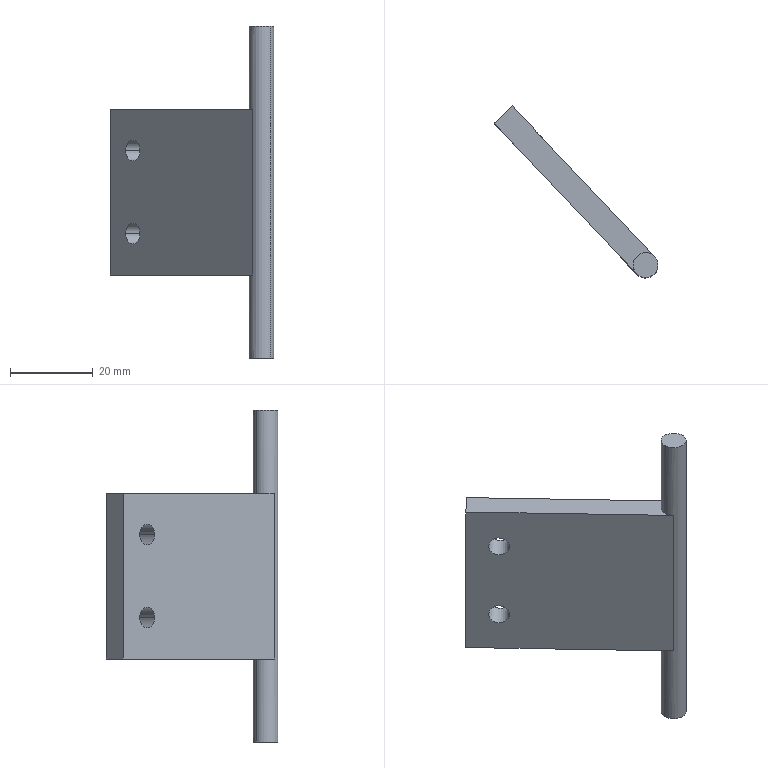Component | SolidWorks | ClampingMechanism-1_ConnectingPinAxis-1 | 1 solid | 13 faces | box 39.51 x 41.41 x 80 mm | volume 13461 mm3 | plane 7 | cylinder 6 | commonest cylinder face diameters 5 x4 6 x2
build123d program:
from build123d import *

# Parameters (mm, degrees)
SKETCH1_R           = 3
BOSS_EXTRUDE1_DEPTH = 40
SKETCH2_W           = 50
SKETCH2_H           = 6
BOSS_EXTRUDE2_DEPTH = 20
SKETCH3_R           = 2.5
CUT_EXTRUDE1_DEPTH  = 10


with BuildPart() as part:
    # Sketch1 → Boss-Extrude1 (new, symmetric)
    with BuildSketch(Plane.XY):
        Circle(SKETCH1_R)
    extrude(amount=BOSS_EXTRUDE1_DEPTH, both=True)

    # Sketch2 → Boss-Extrude2 (add, symmetric)
    with BuildSketch(Plane.XY):
        with Locations((25, 0)):
            Rectangle(SKETCH2_W, SKETCH2_H)
    extrude(amount=BOSS_EXTRUDE2_DEPTH, both=True)

    # Sketch3 → Cut-Extrude1 (cut)
    with BuildSketch(Plane(origin=(0, 3, 0), x_dir=(1, 0, 0), z_dir=(0, 1, 0))):
        with Locations(Location((42, 10, 0), (0, 0, 180))):
            Circle(SKETCH3_R)
        with Locations(Location((42, -10, 0), (0, 0, 180))):
            Circle(SKETCH3_R)
    extrude(amount=-CUT_EXTRUDE1_DEPTH, mode=Mode.SUBTRACT)


solid = part.part

# Placed as in the assembly
solid = solid.moved(Location((-224.378, -274.355, -542.97), (0, 0, 133.363)))
STEP:
#1=CARTESIAN_POINT('',(-9.951,-9.447,-21.77));
#2=VERTEX_POINT('',#1);
#3=CARTESIAN_POINT('',(-9.816,-9.59,-21.77));
#4=VERTEX_POINT('',#3);
#5=CARTESIAN_POINT('',(-9.883,-9.518,-21.77));
#6=DIRECTION('',(-0.727,-0.6866,0.));
#7=DIRECTION('',(0.6866,-0.727,0.));
#8=AXIS2_PLACEMENT_3D('',#5,#6,#7);
#9=CIRCLE('',#8,0.09843);
#10=EDGE_CURVE('',#2,#4,#9,.T.);
#11=ORIENTED_EDGE('',*,*,#10,.F.);
#12=CARTESIAN_POINT('',(-10.123,-9.609,-21.77));
#13=VERTEX_POINT('',#12);
#14=CARTESIAN_POINT('',(-9.836,-9.338,-21.77));
#15=DIRECTION('',(-0.727,-0.6866,0.));
#16=VECTOR('',#15,39.37);
#17=LINE('',#14,#16);
#18=EDGE_CURVE('',#2,#13,#17,.T.);
#19=ORIENTED_EDGE('',*,*,#18,.T.);
#20=CARTESIAN_POINT('',(-9.987,-9.752,-21.77));
#21=VERTEX_POINT('',#20);
#22=CARTESIAN_POINT('',(-10.055,-9.68,-21.77));
#23=DIRECTION('',(-0.727,-0.6866,0.));
#24=DIRECTION('',(0.6866,-0.727,0.));
#25=AXIS2_PLACEMENT_3D('',#22,#23,#24);
#26=CIRCLE('',#25,0.09843);
#27=EDGE_CURVE('',#13,#21,#26,.T.);
#28=ORIENTED_EDGE('',*,*,#27,.T.);
#29=CARTESIAN_POINT('',(-9.701,-9.482,-21.77));
#30=DIRECTION('',(-0.727,-0.6866,0.));
#31=VECTOR('',#30,39.37);
#32=LINE('',#29,#31);
#33=EDGE_CURVE('',#4,#21,#32,.T.);
#34=ORIENTED_EDGE('',*,*,#33,.F.);
#35=EDGE_LOOP('',(#11,#19,#28,#34));
#36=FACE_OUTER_BOUND('',#35,.T.);
#37=CARTESIAN_POINT('',(-9.769,-9.41,-21.77));
#38=DIRECTION('',(-0.727,-0.6866,0.));
#39=DIRECTION('',(0.6866,-0.727,0.));
#40=AXIS2_PLACEMENT_3D('',#37,#38,#39);
#41=CYLINDRICAL_SURFACE('',#40,0.09843);
#42=ADVANCED_FACE('',(#36),#41,.F.);
#43=CARTESIAN_POINT('',(-9.951,-9.447,-20.983));
#44=VERTEX_POINT('',#43);
#45=CARTESIAN_POINT('',(-9.816,-9.59,-20.983));
#46=VERTEX_POINT('',#45);
#47=CARTESIAN_POINT('',(-9.883,-9.518,-20.983));
#48=DIRECTION('',(-0.727,-0.6866,0.));
#49=DIRECTION('',(0.6866,-0.727,0.));
#50=AXIS2_PLACEMENT_3D('',#47,#48,#49);
#51=CIRCLE('',#50,0.09843);
#52=EDGE_CURVE('',#44,#46,#51,.T.);
#53=ORIENTED_EDGE('',*,*,#52,.F.);
#54=CARTESIAN_POINT('',(-10.123,-9.609,-20.983));
#55=VERTEX_POINT('',#54);
#56=CARTESIAN_POINT('',(-9.836,-9.338,-20.983));
#57=DIRECTION('',(-0.727,-0.6866,0.));
#58=VECTOR('',#57,39.37);
#59=LINE('',#56,#58);
#60=EDGE_CURVE('',#44,#55,#59,.T.);
#61=ORIENTED_EDGE('',*,*,#60,.T.);
#62=CARTESIAN_POINT('',(-9.987,-9.752,-20.983));
#63=VERTEX_POINT('',#62);
#64=CARTESIAN_POINT('',(-10.055,-9.68,-20.983));
#65=DIRECTION('',(-0.727,-0.6866,0.));
#66=DIRECTION('',(0.6866,-0.727,0.));
#67=AXIS2_PLACEMENT_3D('',#64,#65,#66);
#68=CIRCLE('',#67,0.09843);
#69=EDGE_CURVE('',#55,#63,#68,.T.);
#70=ORIENTED_EDGE('',*,*,#69,.T.);
#71=CARTESIAN_POINT('',(-9.701,-9.482,-20.983));
#72=DIRECTION('',(-0.727,-0.6866,0.));
#73=VECTOR('',#72,39.37);
#74=LINE('',#71,#73);
#75=EDGE_CURVE('',#46,#63,#74,.T.);
#76=ORIENTED_EDGE('',*,*,#75,.F.);
#77=EDGE_LOOP('',(#53,#61,#70,#76));
#78=FACE_OUTER_BOUND('',#77,.T.);
#79=CARTESIAN_POINT('',(-9.769,-9.41,-20.983));
#80=DIRECTION('',(-0.727,-0.6866,0.));
#81=DIRECTION('',(0.6866,-0.727,0.));
#82=AXIS2_PLACEMENT_3D('',#79,#80,#81);
#83=CYLINDRICAL_SURFACE('',#82,0.09843);
#84=ADVANCED_FACE('',(#78),#83,.F.);
#85=CARTESIAN_POINT('',(-8.915,-10.716,-19.802));
#86=VERTEX_POINT('',#85);
#87=CARTESIAN_POINT('',(-8.753,-10.887,-19.802));
#88=VERTEX_POINT('',#87);
#89=CARTESIAN_POINT('',(-8.834,-10.801,-19.802));
#90=DIRECTION('',(0.,-0.,1.));
#91=DIRECTION('',(-0.6866,0.727,0.));
#92=AXIS2_PLACEMENT_3D('',#89,#90,#91);
#93=CIRCLE('',#92,0.1181);
#94=EDGE_CURVE('',#86,#88,#93,.T.);
#95=ORIENTED_EDGE('',*,*,#94,.F.);
#96=CARTESIAN_POINT('',(-8.915,-10.716,-20.589));
#97=VERTEX_POINT('',#96);
#98=CARTESIAN_POINT('',(-8.915,-10.716,-19.802));
#99=DIRECTION('',(-0.,0.,-1.));
#100=VECTOR('',#99,39.37);
#101=LINE('',#98,#100);
#102=EDGE_CURVE('',#86,#97,#101,.T.);
#103=ORIENTED_EDGE('',*,*,#102,.T.);
#104=CARTESIAN_POINT('',(-8.92,-10.882,-20.589));
#105=VERTEX_POINT('',#104);
#106=CARTESIAN_POINT('',(-8.834,-10.801,-20.589));
#107=DIRECTION('',(-0.,0.,-1.));
#108=DIRECTION('',(0.6866,-0.727,0.));
#109=AXIS2_PLACEMENT_3D('',#106,#107,#108);
#110=CIRCLE('',#109,0.1181);
#111=EDGE_CURVE('',#105,#97,#110,.T.);
#112=ORIENTED_EDGE('',*,*,#111,.F.);
#113=CARTESIAN_POINT('',(-8.92,-10.882,-22.164));
#114=VERTEX_POINT('',#113);
#115=CARTESIAN_POINT('',(-8.92,-10.882,-20.589));
#116=DIRECTION('',(-0.,0.,-1.));
#117=VECTOR('',#116,39.37);
#118=LINE('',#115,#117);
#119=EDGE_CURVE('',#105,#114,#118,.T.);
#120=ORIENTED_EDGE('',*,*,#119,.T.);
#121=CARTESIAN_POINT('',(-8.915,-10.716,-22.164));
#122=VERTEX_POINT('',#121);
#123=CARTESIAN_POINT('',(-8.834,-10.801,-22.164));
#124=DIRECTION('',(-0.,0.,-1.));
#125=DIRECTION('',(0.6866,-0.727,0.));
#126=AXIS2_PLACEMENT_3D('',#123,#124,#125);
#127=CIRCLE('',#126,0.1181);
#128=EDGE_CURVE('',#114,#122,#127,.T.);
#129=ORIENTED_EDGE('',*,*,#128,.T.);
#130=CARTESIAN_POINT('',(-8.915,-10.716,-22.952));
#131=VERTEX_POINT('',#130);
#132=CARTESIAN_POINT('',(-8.915,-10.716,-19.802));
#133=DIRECTION('',(-0.,0.,-1.));
#134=VECTOR('',#133,39.37);
#135=LINE('',#132,#134);
#136=EDGE_CURVE('',#122,#131,#135,.T.);
#137=ORIENTED_EDGE('',*,*,#136,.T.);
#138=CARTESIAN_POINT('',(-8.753,-10.887,-22.952));
#139=VERTEX_POINT('',#138);
#140=CARTESIAN_POINT('',(-8.834,-10.801,-22.952));
#141=DIRECTION('',(0.,-0.,1.));
#142=DIRECTION('',(-0.6866,0.727,0.));
#143=AXIS2_PLACEMENT_3D('',#140,#141,#142);
#144=CIRCLE('',#143,0.1181);
#145=EDGE_CURVE('',#131,#139,#144,.T.);
#146=ORIENTED_EDGE('',*,*,#145,.T.);
#147=CARTESIAN_POINT('',(-8.753,-10.887,-19.802));
#148=DIRECTION('',(-0.,0.,-1.));
#149=VECTOR('',#148,39.37);
#150=LINE('',#147,#149);
#151=EDGE_CURVE('',#88,#139,#150,.T.);
#152=ORIENTED_EDGE('',*,*,#151,.F.);
#153=EDGE_LOOP('',(#95,#103,#112,#120,#129,#137,#146,#152));
#154=FACE_OUTER_BOUND('',#153,.T.);
#155=CARTESIAN_POINT('',(-8.834,-10.801,-19.802));
#156=DIRECTION('',(-0.,0.,-1.));
#157=DIRECTION('',(0.6866,-0.727,0.));
#158=AXIS2_PLACEMENT_3D('',#155,#156,#157);
#159=CYLINDRICAL_SURFACE('',#158,0.1181);
#160=ADVANCED_FACE('',(#154),#159,.T.);
#161=ORIENTED_EDGE('',*,*,#102,.F.);
#162=CARTESIAN_POINT('',(-8.834,-10.801,-19.802));
#163=DIRECTION('',(0.,-0.,1.));
#164=DIRECTION('',(-0.6866,0.727,0.));
#165=AXIS2_PLACEMENT_3D('',#162,#163,#164);
#166=CIRCLE('',#165,0.1181);
#167=EDGE_CURVE('',#88,#86,#166,.T.);
#168=ORIENTED_EDGE('',*,*,#167,.F.);
#169=ORIENTED_EDGE('',*,*,#151,.T.);
#170=CARTESIAN_POINT('',(-8.834,-10.801,-22.952));
#171=DIRECTION('',(0.,-0.,1.));
#172=DIRECTION('',(-0.6866,0.727,0.));
#173=AXIS2_PLACEMENT_3D('',#170,#171,#172);
#174=CIRCLE('',#173,0.1181);
#175=EDGE_CURVE('',#139,#131,#174,.T.);
#176=ORIENTED_EDGE('',*,*,#175,.T.);
#177=ORIENTED_EDGE('',*,*,#136,.F.);
#178=CARTESIAN_POINT('',(-8.748,-10.72,-22.164));
#179=VERTEX_POINT('',#178);
#180=CARTESIAN_POINT('',(-8.834,-10.801,-22.164));
#181=DIRECTION('',(-0.,0.,-1.));
#182=DIRECTION('',(0.6866,-0.727,0.));
#183=AXIS2_PLACEMENT_3D('',#180,#181,#182);
#184=CIRCLE('',#183,0.1181);
#185=EDGE_CURVE('',#122,#179,#184,.T.);
#186=ORIENTED_EDGE('',*,*,#185,.T.);
#187=CARTESIAN_POINT('',(-8.748,-10.72,-20.589));
#188=VERTEX_POINT('',#187);
#189=CARTESIAN_POINT('',(-8.748,-10.72,-20.589));
#190=DIRECTION('',(-0.,0.,-1.));
#191=VECTOR('',#190,39.37);
#192=LINE('',#189,#191);
#193=EDGE_CURVE('',#188,#179,#192,.T.);
#194=ORIENTED_EDGE('',*,*,#193,.F.);
#195=CARTESIAN_POINT('',(-8.834,-10.801,-20.589));
#196=DIRECTION('',(-0.,0.,-1.));
#197=DIRECTION('',(0.6866,-0.727,0.));
#198=AXIS2_PLACEMENT_3D('',#195,#196,#197);
#199=CIRCLE('',#198,0.1181);
#200=EDGE_CURVE('',#97,#188,#199,.T.);
#201=ORIENTED_EDGE('',*,*,#200,.F.);
#202=EDGE_LOOP('',(#161,#168,#169,#176,#177,#186,#194,#201));
#203=FACE_OUTER_BOUND('',#202,.T.);
#204=CARTESIAN_POINT('',(-8.834,-10.801,-19.802));
#205=DIRECTION('',(-0.,0.,-1.));
#206=DIRECTION('',(0.6866,-0.727,0.));
#207=AXIS2_PLACEMENT_3D('',#204,#205,#206);
#208=CYLINDRICAL_SURFACE('',#207,0.1181);
#209=ADVANCED_FACE('',(#203),#208,.T.);
#210=ORIENTED_EDGE('',*,*,#167,.T.);
#211=ORIENTED_EDGE('',*,*,#94,.T.);
#212=EDGE_LOOP('',(#210,#211));
#213=FACE_OUTER_BOUND('',#212,.T.);
#214=CARTESIAN_POINT('',(-8.834,-10.801,-19.802));
#215=DIRECTION('',(0.,-0.,1.));
#216=DIRECTION('',(-0.6866,0.727,0.));
#217=AXIS2_PLACEMENT_3D('',#214,#215,#216);
#218=PLANE('',#217);
#219=ADVANCED_FACE('',(#213),#218,.T.);
#220=ORIENTED_EDGE('',*,*,#175,.F.);
#221=ORIENTED_EDGE('',*,*,#145,.F.);
#222=EDGE_LOOP('',(#220,#221));
#223=FACE_OUTER_BOUND('',#222,.T.);
#224=CARTESIAN_POINT('',(-8.834,-10.801,-22.952));
#225=DIRECTION('',(0.,-0.,1.));
#226=DIRECTION('',(-0.6866,0.727,0.));
#227=AXIS2_PLACEMENT_3D('',#224,#225,#226);
#228=PLANE('',#227);
#229=ADVANCED_FACE('',(#223),#228,.F.);
#230=CARTESIAN_POINT('',(-10.055,-9.68,-21.77));
#231=DIRECTION('',(-0.727,-0.6866,0.));
#232=DIRECTION('',(0.6866,-0.727,0.));
#233=AXIS2_PLACEMENT_3D('',#230,#231,#232);
#234=CIRCLE('',#233,0.09843);
#235=EDGE_CURVE('',#21,#13,#234,.T.);
#236=ORIENTED_EDGE('',*,*,#235,.F.);
#237=ORIENTED_EDGE('',*,*,#27,.F.);
#238=EDGE_LOOP('',(#236,#237));
#239=FACE_BOUND('',#238,.T.);
#240=CARTESIAN_POINT('',(-10.055,-9.68,-20.983));
#241=DIRECTION('',(-0.727,-0.6866,0.));
#242=DIRECTION('',(0.6866,-0.727,0.));
#243=AXIS2_PLACEMENT_3D('',#240,#241,#242);
#244=CIRCLE('',#243,0.09843);
#245=EDGE_CURVE('',#63,#55,#244,.T.);
#246=ORIENTED_EDGE('',*,*,#245,.F.);
#247=ORIENTED_EDGE('',*,*,#69,.F.);
#248=EDGE_LOOP('',(#246,#247));
#249=FACE_BOUND('',#248,.T.);
#250=CARTESIAN_POINT('',(-10.271,-9.451,-22.164));
#251=VERTEX_POINT('',#250);
#252=CARTESIAN_POINT('',(-8.92,-10.882,-22.164));
#253=DIRECTION('',(0.6866,-0.727,-0.));
#254=VECTOR('',#253,39.37);
#255=LINE('',#252,#254);
#256=EDGE_CURVE('',#251,#114,#255,.T.);
#257=ORIENTED_EDGE('',*,*,#256,.T.);
#258=ORIENTED_EDGE('',*,*,#119,.F.);
#259=CARTESIAN_POINT('',(-10.271,-9.451,-20.589));
#260=VERTEX_POINT('',#259);
#261=CARTESIAN_POINT('',(-8.92,-10.882,-20.589));
#262=DIRECTION('',(0.6866,-0.727,-0.));
#263=VECTOR('',#262,39.37);
#264=LINE('',#261,#263);
#265=EDGE_CURVE('',#260,#105,#264,.T.);
#266=ORIENTED_EDGE('',*,*,#265,.F.);
#267=CARTESIAN_POINT('',(-10.271,-9.451,-20.589));
#268=DIRECTION('',(-0.,0.,-1.));
#269=VECTOR('',#268,39.37);
#270=LINE('',#267,#269);
#271=EDGE_CURVE('',#260,#251,#270,.T.);
#272=ORIENTED_EDGE('',*,*,#271,.T.);
#273=EDGE_LOOP('',(#257,#258,#266,#272));
#274=FACE_OUTER_BOUND('',#273,.T.);
#275=CARTESIAN_POINT('',(-8.92,-10.882,-20.589));
#276=DIRECTION('',(0.727,0.6866,-0.));
#277=DIRECTION('',(-0.6866,0.727,0.));
#278=AXIS2_PLACEMENT_3D('',#275,#276,#277);
#279=PLANE('',#278);
#280=ADVANCED_FACE('',(#239,#249,#274),#279,.F.);
#281=CARTESIAN_POINT('',(-9.883,-9.518,-21.77));
#282=DIRECTION('',(-0.727,-0.6866,0.));
#283=DIRECTION('',(0.6866,-0.727,0.));
#284=AXIS2_PLACEMENT_3D('',#281,#282,#283);
#285=CIRCLE('',#284,0.09843);
#286=EDGE_CURVE('',#4,#2,#285,.T.);
#287=ORIENTED_EDGE('',*,*,#286,.T.);
#288=ORIENTED_EDGE('',*,*,#10,.T.);
#289=EDGE_LOOP('',(#287,#288));
#290=FACE_BOUND('',#289,.T.);
#291=CARTESIAN_POINT('',(-9.883,-9.518,-20.983));
#292=DIRECTION('',(-0.727,-0.6866,0.));
#293=DIRECTION('',(0.6866,-0.727,0.));
#294=AXIS2_PLACEMENT_3D('',#291,#292,#293);
#295=CIRCLE('',#294,0.09843);
#296=EDGE_CURVE('',#46,#44,#295,.T.);
#297=ORIENTED_EDGE('',*,*,#296,.T.);
#298=ORIENTED_EDGE('',*,*,#52,.T.);
#299=EDGE_LOOP('',(#297,#298));
#300=FACE_BOUND('',#299,.T.);
#301=CARTESIAN_POINT('',(-10.1,-9.289,-22.164));
#302=VERTEX_POINT('',#301);
#303=CARTESIAN_POINT('',(-8.748,-10.72,-22.164));
#304=DIRECTION('',(-0.6866,0.727,0.));
#305=VECTOR('',#304,39.37);
#306=LINE('',#303,#305);
#307=EDGE_CURVE('',#179,#302,#306,.T.);
#308=ORIENTED_EDGE('',*,*,#307,.T.);
#309=CARTESIAN_POINT('',(-10.1,-9.289,-20.589));
#310=VERTEX_POINT('',#309);
#311=CARTESIAN_POINT('',(-10.1,-9.289,-20.589));
#312=DIRECTION('',(-0.,0.,-1.));
#313=VECTOR('',#312,39.37);
#314=LINE('',#311,#313);
#315=EDGE_CURVE('',#310,#302,#314,.T.);
#316=ORIENTED_EDGE('',*,*,#315,.F.);
#317=CARTESIAN_POINT('',(-8.748,-10.72,-20.589));
#318=DIRECTION('',(-0.6866,0.727,0.));
#319=VECTOR('',#318,39.37);
#320=LINE('',#317,#319);
#321=EDGE_CURVE('',#188,#310,#320,.T.);
#322=ORIENTED_EDGE('',*,*,#321,.F.);
#323=ORIENTED_EDGE('',*,*,#193,.T.);
#324=EDGE_LOOP('',(#308,#316,#322,#323));
#325=FACE_OUTER_BOUND('',#324,.T.);
#326=CARTESIAN_POINT('',(-8.748,-10.72,-20.589));
#327=DIRECTION('',(-0.727,-0.6866,0.));
#328=DIRECTION('',(0.6866,-0.727,-0.));
#329=AXIS2_PLACEMENT_3D('',#326,#327,#328);
#330=PLANE('',#329);
#331=ADVANCED_FACE('',(#290,#300,#325),#330,.F.);
#332=CARTESIAN_POINT('',(-10.271,-9.451,-22.164));
#333=DIRECTION('',(-0.727,-0.6866,0.));
#334=VECTOR('',#333,39.37);
#335=LINE('',#332,#334);
#336=EDGE_CURVE('',#302,#251,#335,.T.);
#337=ORIENTED_EDGE('',*,*,#336,.T.);
#338=ORIENTED_EDGE('',*,*,#271,.F.);
#339=CARTESIAN_POINT('',(-10.271,-9.451,-20.589));
#340=DIRECTION('',(-0.727,-0.6866,0.));
#341=VECTOR('',#340,39.37);
#342=LINE('',#339,#341);
#343=EDGE_CURVE('',#310,#260,#342,.T.);
#344=ORIENTED_EDGE('',*,*,#343,.F.);
#345=ORIENTED_EDGE('',*,*,#315,.T.);
#346=EDGE_LOOP('',(#337,#338,#344,#345));
#347=FACE_OUTER_BOUND('',#346,.T.);
#348=CARTESIAN_POINT('',(-10.271,-9.451,-20.589));
#349=DIRECTION('',(0.6866,-0.727,-0.));
#350=DIRECTION('',(0.,-0.,1.));
#351=AXIS2_PLACEMENT_3D('',#348,#349,#350);
#352=PLANE('',#351);
#353=ADVANCED_FACE('',(#347),#352,.F.);
#354=ORIENTED_EDGE('',*,*,#265,.T.);
#355=ORIENTED_EDGE('',*,*,#111,.T.);
#356=ORIENTED_EDGE('',*,*,#200,.T.);
#357=ORIENTED_EDGE('',*,*,#321,.T.);
#358=ORIENTED_EDGE('',*,*,#343,.T.);
#359=EDGE_LOOP('',(#354,#355,#356,#357,#358));
#360=FACE_OUTER_BOUND('',#359,.T.);
#361=CARTESIAN_POINT('',(-8.834,-10.801,-20.589));
#362=DIRECTION('',(-0.,0.,-1.));
#363=DIRECTION('',(0.6866,-0.727,-0.));
#364=AXIS2_PLACEMENT_3D('',#361,#362,#363);
#365=PLANE('',#364);
#366=ADVANCED_FACE('',(#360),#365,.F.);
#367=ORIENTED_EDGE('',*,*,#128,.F.);
#368=ORIENTED_EDGE('',*,*,#256,.F.);
#369=ORIENTED_EDGE('',*,*,#336,.F.);
#370=ORIENTED_EDGE('',*,*,#307,.F.);
#371=ORIENTED_EDGE('',*,*,#185,.F.);
#372=EDGE_LOOP('',(#367,#368,#369,#370,#371));
#373=FACE_OUTER_BOUND('',#372,.T.);
#374=CARTESIAN_POINT('',(-8.834,-10.801,-22.164));
#375=DIRECTION('',(-0.,0.,-1.));
#376=DIRECTION('',(0.6866,-0.727,-0.));
#377=AXIS2_PLACEMENT_3D('',#374,#375,#376);
#378=PLANE('',#377);
#379=ADVANCED_FACE('',(#373),#378,.T.);
#380=ORIENTED_EDGE('',*,*,#60,.F.);
#381=ORIENTED_EDGE('',*,*,#296,.F.);
#382=ORIENTED_EDGE('',*,*,#75,.T.);
#383=ORIENTED_EDGE('',*,*,#245,.T.);
#384=EDGE_LOOP('',(#380,#381,#382,#383));
#385=FACE_OUTER_BOUND('',#384,.T.);
#386=CARTESIAN_POINT('',(-9.769,-9.41,-20.983));
#387=DIRECTION('',(-0.727,-0.6866,0.));
#388=DIRECTION('',(0.6866,-0.727,0.));
#389=AXIS2_PLACEMENT_3D('',#386,#387,#388);
#390=CYLINDRICAL_SURFACE('',#389,0.09843);
#391=ADVANCED_FACE('',(#385),#390,.F.);
#392=ORIENTED_EDGE('',*,*,#18,.F.);
#393=ORIENTED_EDGE('',*,*,#286,.F.);
#394=ORIENTED_EDGE('',*,*,#33,.T.);
#395=ORIENTED_EDGE('',*,*,#235,.T.);
#396=EDGE_LOOP('',(#392,#393,#394,#395));
#397=FACE_OUTER_BOUND('',#396,.T.);
#398=CARTESIAN_POINT('',(-9.769,-9.41,-21.77));
#399=DIRECTION('',(-0.727,-0.6866,0.));
#400=DIRECTION('',(0.6866,-0.727,0.));
#401=AXIS2_PLACEMENT_3D('',#398,#399,#400);
#402=CYLINDRICAL_SURFACE('',#401,0.09843);
#403=ADVANCED_FACE('',(#397),#402,.F.);
#404=CLOSED_SHELL('',(#42,#84,#160,#209,#219,#229,#280,#331,#353,#366,#379,#391,#403));
#405=MANIFOLD_SOLID_BREP('',#404);
#406=CARTESIAN_POINT('',(0.,0.,0.));
#407=DIRECTION('',(0.,0.,1.));
#408=DIRECTION('',(1.,0.,0.));
#409=AXIS2_PLACEMENT_3D('',#406,#407,#408);
#410=(LENGTH_UNIT()NAMED_UNIT(*)SI_UNIT($,.METRE.));
#411=LENGTH_MEASURE_WITH_UNIT(LENGTH_MEASURE(0.0254),#410);
#412=DIMENSIONAL_EXPONENTS(1.,0.,0.,0.,0.,0.,0.);
#413=(CONVERSION_BASED_UNIT('',#411)LENGTH_UNIT()NAMED_UNIT(#412));
#414=UNCERTAINTY_MEASURE_WITH_UNIT(LENGTH_MEASURE(0.00001),#413,'','');
#415=(NAMED_UNIT(*)PLANE_ANGLE_UNIT()SI_UNIT($,.RADIAN.));
#416=(NAMED_UNIT(*)SI_UNIT($,.STERADIAN.)SOLID_ANGLE_UNIT());
#417=(GEOMETRIC_REPRESENTATION_CONTEXT(3)GLOBAL_UNCERTAINTY_ASSIGNED_CONTEXT((#414))GLOBAL_UNIT_ASSIGNED_CONTEXT((#413,#415,#416))REPRESENTATION_CONTEXT('',''));
#418=ADVANCED_BREP_SHAPE_REPRESENTATION('',(#405,#409),#417);
#419=COLOUR_RGB('',0.7922,0.8196,0.9333);
#420=FILL_AREA_STYLE_COLOUR('',#419);
#421=FILL_AREA_STYLE('',(#420));
#422=SURFACE_STYLE_FILL_AREA(#421);
#423=SURFACE_SIDE_STYLE('',(#422));
#424=SURFACE_STYLE_USAGE(.BOTH.,#423);
#425=PRESENTATION_STYLE_ASSIGNMENT((#424));
#426=STYLED_ITEM('',(#425),#405);
#427=PRESENTATION_LAYER_ASSIGNMENT('','',(#426));
#428=(LENGTH_UNIT()NAMED_UNIT(*)SI_UNIT($,.METRE.));
#429=LENGTH_MEASURE_WITH_UNIT(LENGTH_MEASURE(0.0254),#428);
#430=DIMENSIONAL_EXPONENTS(1.,0.,0.,0.,0.,0.,0.);
#431=(CONVERSION_BASED_UNIT('',#429)LENGTH_UNIT()NAMED_UNIT(#430));
#432=UNCERTAINTY_MEASURE_WITH_UNIT(LENGTH_MEASURE(0.00001),#431,'','');
#433=(NAMED_UNIT(*)PLANE_ANGLE_UNIT()SI_UNIT($,.RADIAN.));
#434=(NAMED_UNIT(*)SI_UNIT($,.STERADIAN.)SOLID_ANGLE_UNIT());
#435=(GEOMETRIC_REPRESENTATION_CONTEXT(3)GLOBAL_UNCERTAINTY_ASSIGNED_CONTEXT((#432))GLOBAL_UNIT_ASSIGNED_CONTEXT((#431,#433,#434))REPRESENTATION_CONTEXT('',''));
#436=MECHANICAL_DESIGN_GEOMETRIC_PRESENTATION_REPRESENTATION('',(#426),#435);